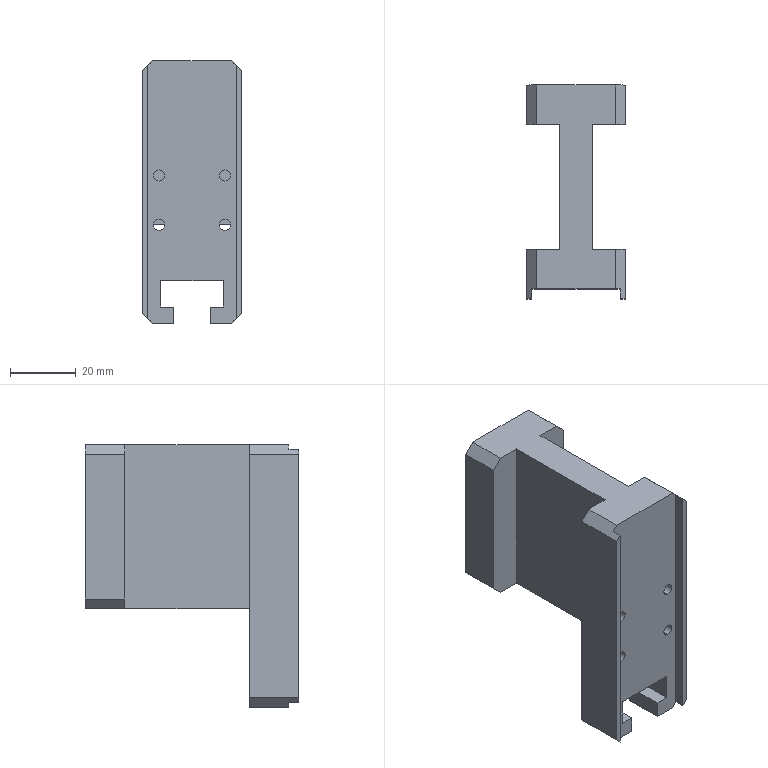Component | SolidWorks | ThirdGenerationFour-sidedLabelingFeedingSliderConnectionPlate-1 | 1 solid | 46 faces | box 30 x 65 x 80 mm | volume 62845 mm3 | plane 34 | cylinder 10 | cone 2 | commonest cylinder face diameters 3.4 x8 4.2 x2
build123d program:
from build123d import *

# Parameters (mm, degrees)
SKETCH1_W                      = 80
SKETCH1_H                      = 30
BOSS_EXTRUDE1_DEPTH            = 32.5
SKETCH2_W                      = 140.082
SKETCH2_H                      = 27
CUT_EXTRUDE1_DEPTH             = 3
F_3_4_3_4_DIAMETER_HOLE1_D     = 3.4
F_3_4_3_4_DIAMETER_HOLE1_DEPTH = 20
F_3_4_3_4_DIAMETER_HOLE1_TIP   = 1.021
SKETCH5_W                      = 10
SKETCH5_H                      = 11
CUT_EXTRUDE2_DEPTH             = 78.782
SKETCH6_W                      = 8
SKETCH6_H                      = 19
CUT_EXTRUDE3_DEPTH             = 78.782
M5_TAPPED_HOLE2_D              = 4.2
M5_TAPPED_HOLE2_DEPTH          = 20
M5_TAPPED_HOLE2_TIP            = 1.262
SKETCH13_W                     = 121.156
SKETCH13_H                     = 38
CUT_EXTRUDE4_DEPTH             = 10
CUT_EXTRUDE5_REACH             = 82.889
SKETCH14_W                     = 57.856
SKETCH14_H                     = 68.267
CHAMFER1_SIZE                  = 3


with BuildPart() as part:
    # Sketch1 → Boss-Extrude1 (new, symmetric)
    with BuildSketch(Plane.XY):
        Rectangle(SKETCH1_W, SKETCH1_H)
    extrude(amount=BOSS_EXTRUDE1_DEPTH, both=True)

    # Sketch2 → Cut-Extrude1 (cut)
    with BuildSketch(Plane.XY.offset(32.5)):
        Rectangle(SKETCH2_W, SKETCH2_H)
    extrude(amount=-CUT_EXTRUDE1_DEPTH, mode=Mode.SUBTRACT)

    # 3.4 _3.4_ Diameter Hole1
    with Locations(Plane(origin=(30.14, -0.2316, 29.5), x_dir=(-1, 0, 0), z_dir=(0, 0, 1))):
        with Locations((25.14, -10.232), (40.14, -10.232), (40.14, 9.768), (25.14, 9.768)):
            Hole(F_3_4_3_4_DIAMETER_HOLE1_D / 2, depth=F_3_4_3_4_DIAMETER_HOLE1_DEPTH)
            with Locations((0, 0, -(F_3_4_3_4_DIAMETER_HOLE1_DEPTH + F_3_4_3_4_DIAMETER_HOLE1_TIP / 2))):  # 118° drill point
                Cone(0, F_3_4_3_4_DIAMETER_HOLE1_D / 2, F_3_4_3_4_DIAMETER_HOLE1_TIP, mode=Mode.SUBTRACT)

    # Sketch5 → Cut-Extrude2 (cut, through all)
    with BuildSketch(Plane(origin=(0, 0, -32.5), x_dir=(-1, 0, 0), z_dir=(0, 0, -1))):
        with Locations((40, 0)):
            Rectangle(SKETCH5_W, SKETCH5_H)
    extrude(amount=-CUT_EXTRUDE2_DEPTH, mode=Mode.SUBTRACT)

    # Sketch6 → Cut-Extrude3 (cut, through all)
    with BuildSketch(Plane(origin=(0, 0, -32.5), x_dir=(-1, 0, 0), z_dir=(0, 0, -1))):
        with Locations((31, 0)):
            Rectangle(SKETCH6_W, SKETCH6_H)
    extrude(amount=-CUT_EXTRUDE3_DEPTH, mode=Mode.SUBTRACT)

    # M5 Tapped Hole2
    with Locations(Plane(origin=(0, 0, -32.5), x_dir=(-1, 0, 0), z_dir=(0, 0, -1))):
        with Locations((-10, 0)):
            Hole(M5_TAPPED_HOLE2_D / 2, depth=M5_TAPPED_HOLE2_DEPTH)
            with Locations((0, 0, -(M5_TAPPED_HOLE2_DEPTH + M5_TAPPED_HOLE2_TIP / 2))):  # 118° drill point
                Cone(0, M5_TAPPED_HOLE2_D / 2, M5_TAPPED_HOLE2_TIP, mode=Mode.SUBTRACT)

    # Sketch13 → Cut-Extrude4 (cut)
    with BuildSketch(Plane.XZ.offset(15)):
        with Locations((8.72, -1.5)):
            Rectangle(SKETCH13_W, SKETCH13_H)
    cut_extrude4 = extrude(amount=-CUT_EXTRUDE4_DEPTH, mode=Mode.SUBTRACT)

    # Mirror1: Cut-Extrude4 across plane
    add(cut_extrude4.mirror(Plane.ZX), mode=Mode.SUBTRACT)

    # Cut-Extrude5: up to this face of the body (flat: up to its plane)
    cut_extrude5_end = Plane(part.part.faces().sort_by_distance((1.689, 10.149, 17.5))[0])
    # Sketch14 → Cut-Extrude5 (cut, up to the picked face)
    with BuildSketch(Plane(origin=(-5.75, 0, -32.5), x_dir=(1, 0, 0), z_dir=(0, 0, 1)), mode=Mode.PRIVATE) as cut_extrude5_sk1:
        with Locations((-33.178, 8.581)):
            Rectangle(SKETCH14_W, SKETCH14_H)
    cut_extrude5_tool1 = split(extrude(cut_extrude5_sk1.sketch, amount=CUT_EXTRUDE5_REACH, mode=Mode.PRIVATE), bisect_by=cut_extrude5_end, keep=Keep.BOTH, mode=Mode.PRIVATE)
    add(cut_extrude5_tool1.solids().sort_by(Axis((-38.928, 8.581, -32.5), (0, 0, 1)))[0], mode=Mode.SUBTRACT)

    # Chamfer1
    chamfer1_edges = [part.edges().sort_by_distance(p)[0] for p in [
        (-40, 15, 25),
        (-40, -15, 25),
        (40, -15, 25),
        (40, -15, -26.5),
        (40, 15, 25),
        (40, 15, -26.5),
        (-10, 15, -26.5),
        (-10, -15, -26.5),
    ]]
    chamfer(chamfer1_edges, length=CHAMFER1_SIZE)


solid = part.part

# Placed as in the assembly
solid = solid.moved(Location((59.473, 6.363, -111.5), (90, 0, 90)))